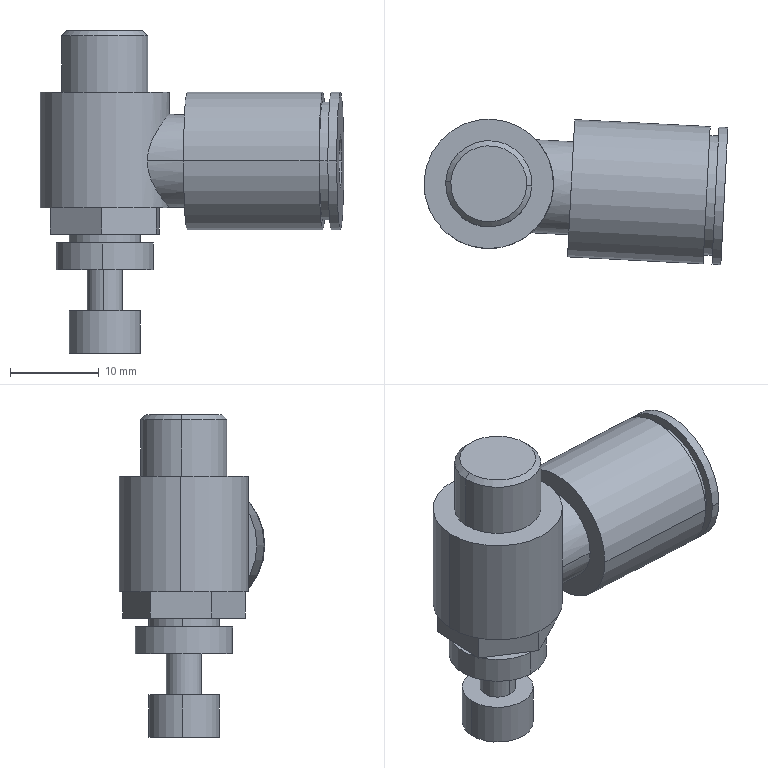Component | SolidWorks | AS2201-01-F06S-1 | 1 solid | 43 faces | volume 6653 mm3 | cylinder 22 | plane 18 | cone 2 | spline 1 | commonest cylinder face diameters 15.5 x4 8 x4 9.73 x2 14.6 x2 10.5 x2 13.5 x2 11 x2 4 x2